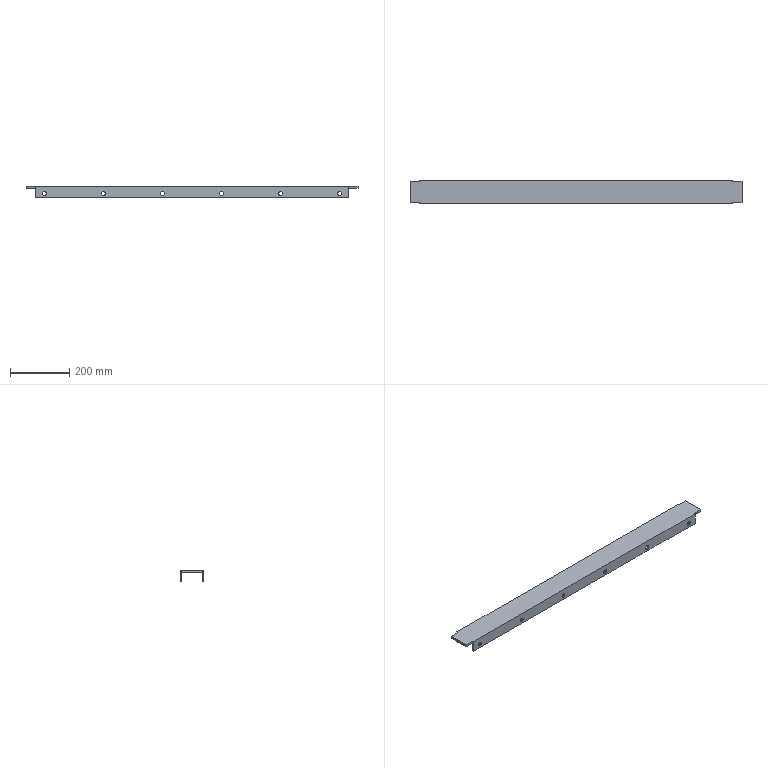Component | SolidWorks | BaseAssembly-1_ChannelSteelAssembly-1_8#ChannelSteel2-1 | 1 solid | 42 faces | box 1124 x 80 x 40 mm | volume 979235 mm3 | cylinder 24 | plane 18 | commonest cylinder face diameters 14 x24
build123d program:
from build123d import *

# Parameters (mm, degrees)
EXTRUDE1_DEPTH     = 1124
SKETCH2_W          = 32
SKETCH2_H          = 32
CUT_EXTRUDE1_DEPTH = 1128.553
SKETCH3_W          = 32
SKETCH3_H          = 4
CUT_EXTRUDE2_DEPTH = 1200
SKETCH4_R          = 7
CUT_EXTRUDE3_DEPTH = 1128.553
LPATTERN1_COUNT    = 6
LPATTERN1_PITCH    = 200


with BuildPart() as part:
    # Sketch1 → Extrude1 (new body)
    with BuildSketch(Plane.XY):
        Polygon((0, 0), (-40, 0), (-40, 80), (0, 80), (0, 76), (-32, 76), (-32, 4), (0, 4), align=None)
    extrude(amount=EXTRUDE1_DEPTH)

    # Sketch2 → Cut-Extrude1 (cut, through all)
    with BuildSketch(Plane(origin=(0, 80, 0), x_dir=(1, 0, 0), z_dir=(0, 1, 0))):
        with Locations((-16, -16)):
            Rectangle(SKETCH2_W, SKETCH2_H)
        with Locations((-16, -1108)):
            Rectangle(SKETCH2_W, SKETCH2_H)
    extrude(amount=-CUT_EXTRUDE1_DEPTH, mode=Mode.SUBTRACT)

    # Sketch3 → Cut-Extrude2 (cut)
    with BuildSketch(Plane(origin=(-32, 0, 0), x_dir=(0, 0, -1), z_dir=(1, 0, 0))):
        with Locations((-1108, 78)):
            Rectangle(SKETCH3_W, SKETCH3_H)
        with Locations((-1108, 2)):
            Rectangle(SKETCH3_W, SKETCH3_H)
        with Locations((-16, 78)):
            Rectangle(SKETCH3_W, SKETCH3_H)
        with Locations((-16, 2)):
            Rectangle(SKETCH3_W, SKETCH3_H)
    extrude(amount=-CUT_EXTRUDE2_DEPTH, mode=Mode.SUBTRACT)

    # Sketch4 → Cut-Extrude3 (cut, through all)
    with BuildSketch(Plane(origin=(0, 80, 0), x_dir=(1, 0, 0), z_dir=(0, 1, 0))):
        with Locations(Location((-15, -1062, 0), (0, 0, 270))):
            Circle(SKETCH4_R)
    cut_extrude3 = extrude(amount=-CUT_EXTRUDE3_DEPTH, mode=Mode.SUBTRACT)

    # LPattern1: Cut-Extrude3 ×6
    with Locations(*[(0, 0, -i * LPATTERN1_PITCH) for i in range(1, LPATTERN1_COUNT)]):
        add(cut_extrude3, mode=Mode.SUBTRACT)


solid = part.part

# Placed as in the assembly
solid = solid.moved(Location((-409.218, -82.9, 360), (0, 90, 0)))